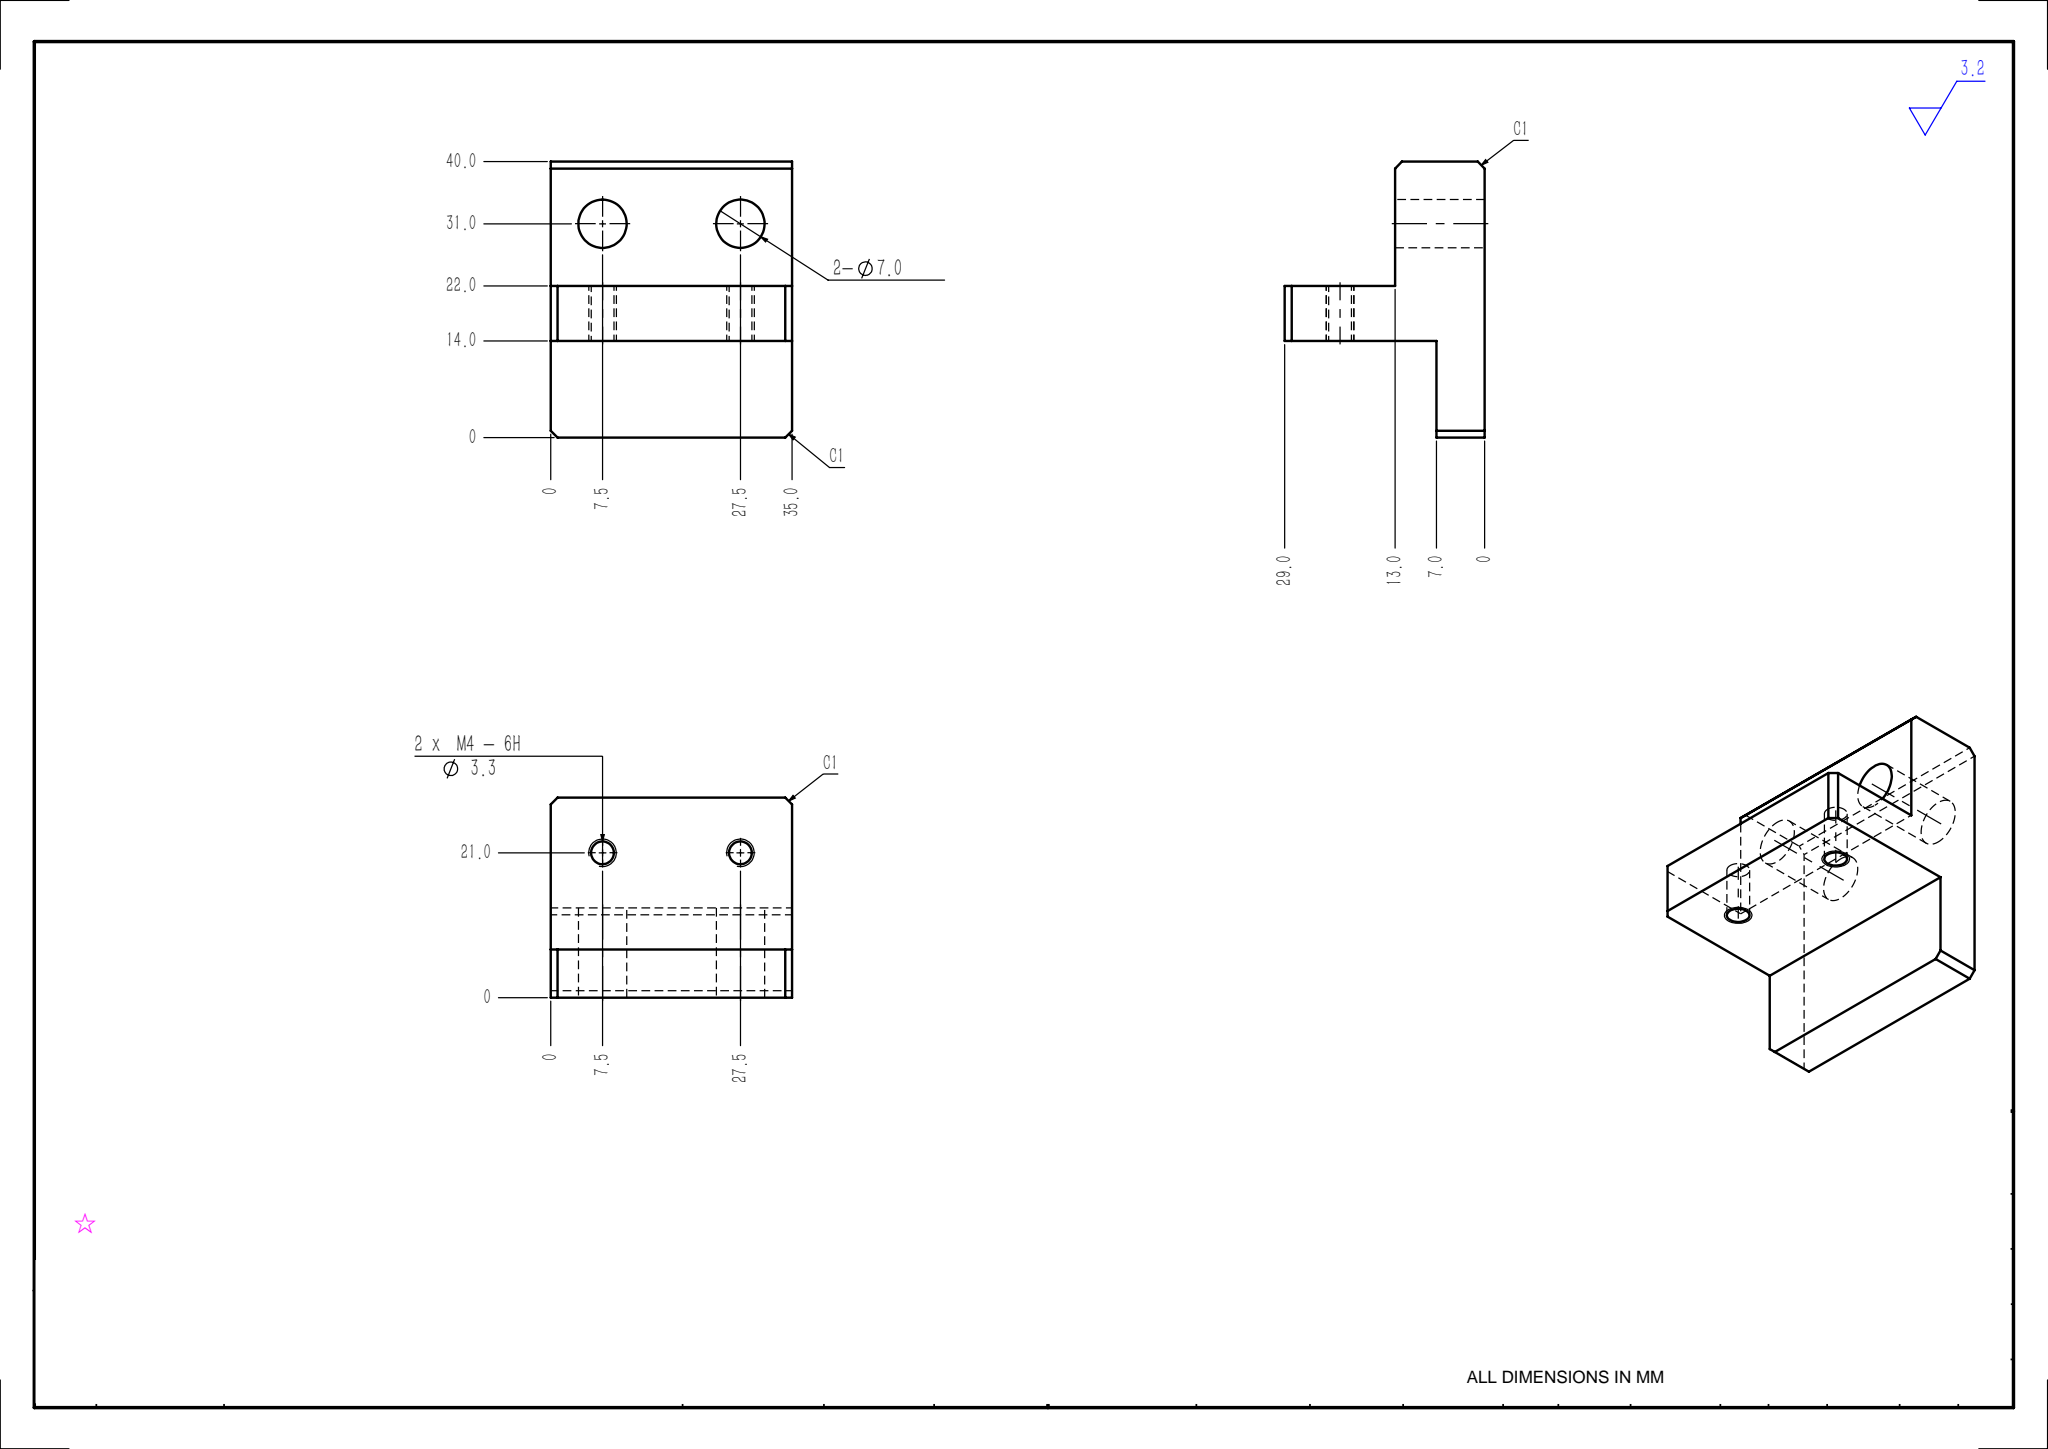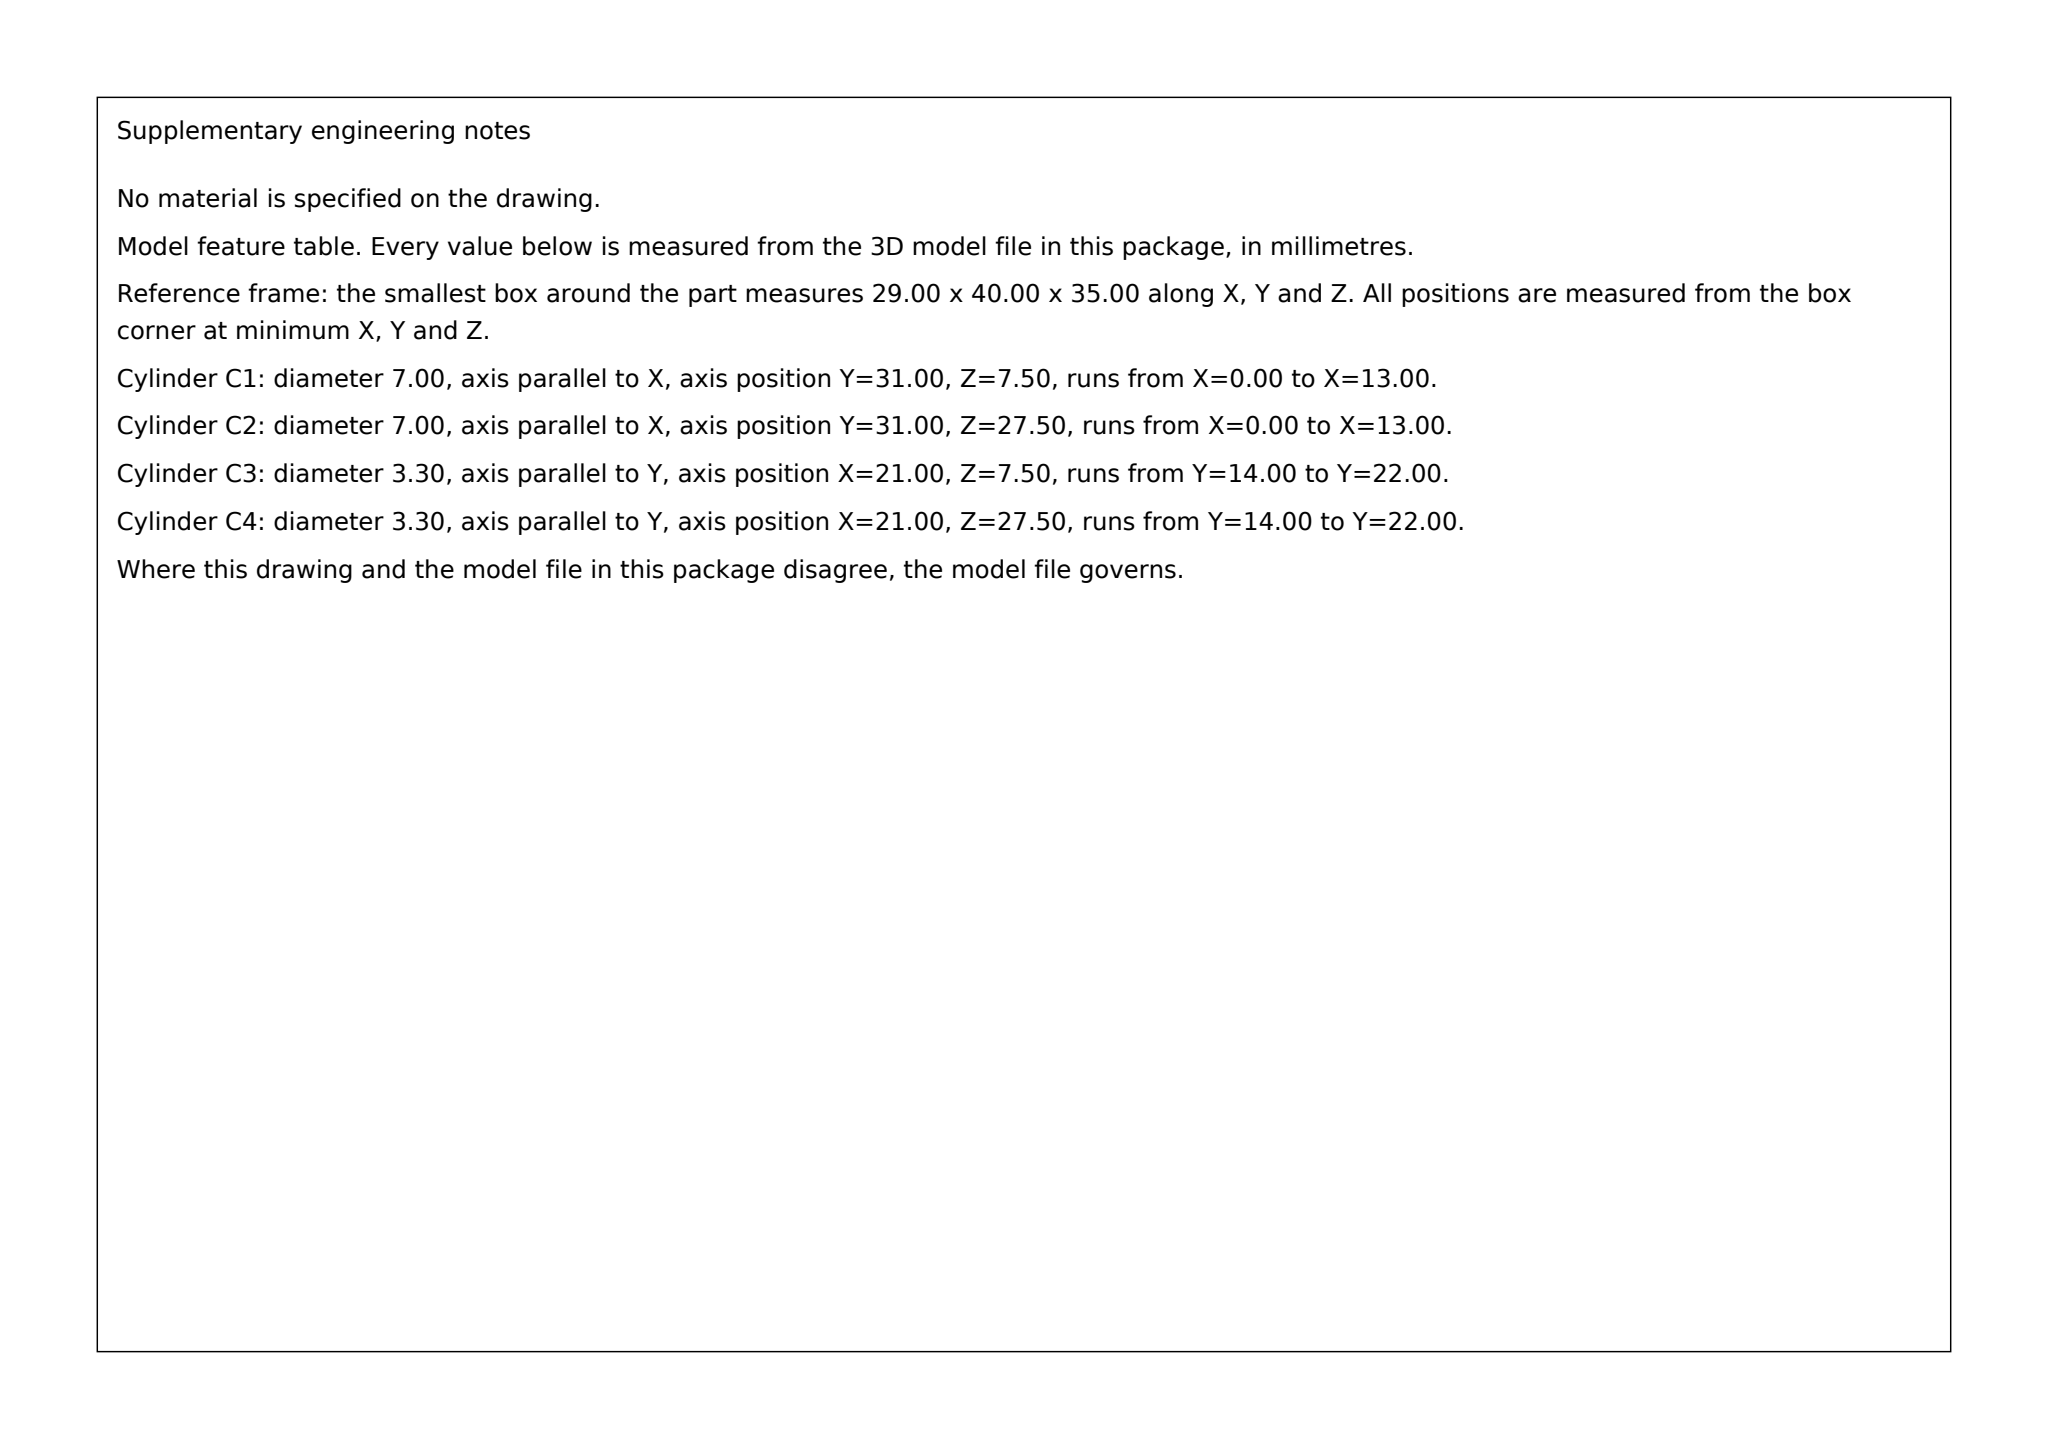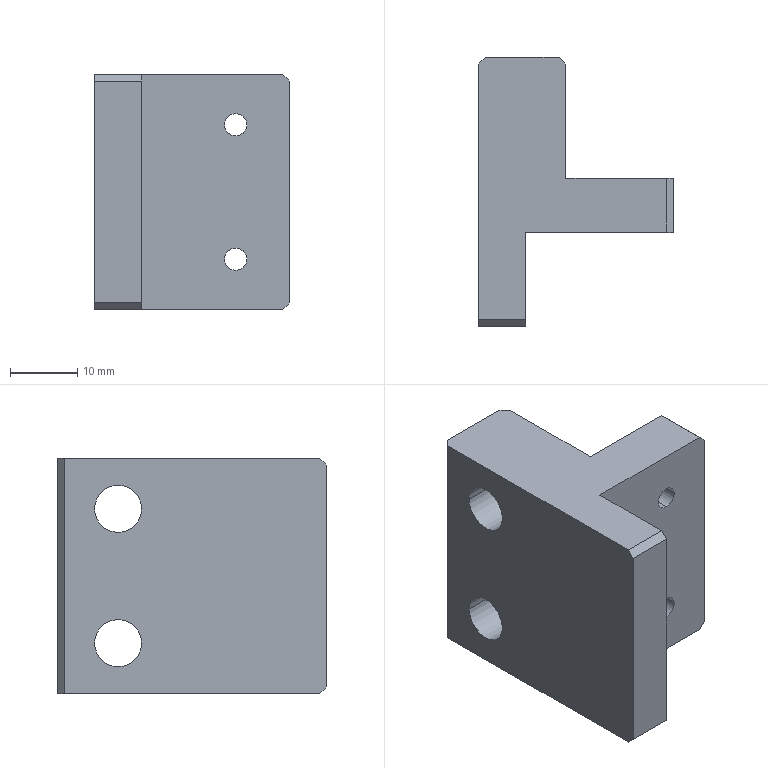Part | SolidWorks | mm | 1 solid | 24 faces | box 29 x 40 x 35 mm | volume 18553 mm3 | plane 16 | cylinder 8 | commonest cylinder face diameters 3.3 x4 7 x4
build123d program:
from build123d import *

# Parameters (mm, degrees)
SKETCH1_W           = 29
SKETCH1_H           = 40
BOSS_EXTRUDE1_DEPTH = 17.5
SKETCH2_W           = 22
SKETCH2_H           = 14
SKETCH2_W_2         = 16
SKETCH2_H_2         = 18
CUT_EXTRUDE1_DEPTH  = 43.84
SKETCH3_R           = 3.5
CUT_EXTRUDE2_DEPTH  = 32.02
M4_TAPPED_HOLE1_D   = 3.3
CHAMFER1_SIZE       = 1


with BuildPart() as part:
    # Sketch1 → Boss-Extrude1 (new, symmetric)
    with BuildSketch(Plane.XY):
        Rectangle(SKETCH1_W, SKETCH1_H)
    extrude(amount=BOSS_EXTRUDE1_DEPTH, both=True)

    # Sketch2 → Cut-Extrude1 (cut, through all)
    with BuildSketch(Plane.XY.offset(17.5)):
        with Locations((3.5, -13)):
            Rectangle(SKETCH2_W, SKETCH2_H)
        with Locations((6.5, 11)):
            Rectangle(SKETCH2_W_2, SKETCH2_H_2)
    extrude(amount=-CUT_EXTRUDE1_DEPTH, mode=Mode.SUBTRACT)

    # Sketch3 → Cut-Extrude2 (cut, through all)
    with BuildSketch(Plane(origin=(-1.5, 0, 0), x_dir=(0, 0, -1), z_dir=(1, 0, 0))):
        with Locations(Location((-10, 11, 0), (0, 0, 90))):
            Circle(SKETCH3_R)
        with Locations(Location((10, 11, 0), (0, 0, 270))):
            Circle(SKETCH3_R)
    extrude(amount=-CUT_EXTRUDE2_DEPTH, mode=Mode.SUBTRACT)

    # M4 Tapped Hole1 (through all)
    with Locations(Plane(origin=(0, -6, 0), x_dir=(-1, 0, 0), z_dir=(0, -1, 0))):
        with Locations((-6.5, 10), (-6.5, -10)):
            Hole(M4_TAPPED_HOLE1_D / 2)

    # Chamfer1
    chamfer1_edges = [part.edges().sort_by_distance(p)[0] for p in [
        (-11, -20, 17.5),
        (14.5, -2, -17.5),
        (14.5, -2, 17.5),
        (-1.5, 20, 0),
        (-11, -20, -17.5),
        (-14.5, 20, 0),
    ]]
    chamfer(chamfer1_edges, length=CHAMFER1_SIZE)


solid = part.part
STEP:
#1=CARTESIAN_POINT('',(6.5,2.,-8.35));
#2=VERTEX_POINT('',#1);
#3=CARTESIAN_POINT('',(6.5,2.,-11.65));
#4=VERTEX_POINT('',#3);
#5=CARTESIAN_POINT('',(6.5,2.,-10.));
#6=DIRECTION('',(0.,-1.,0.));
#7=DIRECTION('',(1.,0.,0.));
#8=AXIS2_PLACEMENT_3D('',#5,#6,#7);
#9=CIRCLE('',#8,1.65);
#10=EDGE_CURVE('',#2,#4,#9,.T.);
#11=ORIENTED_EDGE('',*,*,#10,.F.);
#12=CARTESIAN_POINT('',(6.5,-6.,-8.35));
#13=VERTEX_POINT('',#12);
#14=CARTESIAN_POINT('',(6.5,-6.,-8.35));
#15=DIRECTION('',(0.,-1.,0.));
#16=VECTOR('',#15,1000.);
#17=LINE('',#14,#16);
#18=EDGE_CURVE('',#2,#13,#17,.T.);
#19=ORIENTED_EDGE('',*,*,#18,.T.);
#20=CARTESIAN_POINT('',(6.5,-6.,-11.65));
#21=VERTEX_POINT('',#20);
#22=CARTESIAN_POINT('',(6.5,-6.,-10.));
#23=DIRECTION('',(0.,-1.,0.));
#24=DIRECTION('',(0.,0.,-1.));
#25=AXIS2_PLACEMENT_3D('',#22,#23,#24);
#26=CIRCLE('',#25,1.65);
#27=EDGE_CURVE('',#13,#21,#26,.T.);
#28=ORIENTED_EDGE('',*,*,#27,.T.);
#29=CARTESIAN_POINT('',(6.5,-6.,-11.65));
#30=DIRECTION('',(0.,-1.,0.));
#31=VECTOR('',#30,1000.);
#32=LINE('',#29,#31);
#33=EDGE_CURVE('',#4,#21,#32,.T.);
#34=ORIENTED_EDGE('',*,*,#33,.F.);
#35=EDGE_LOOP('',(#11,#19,#28,#34));
#36=FACE_OUTER_BOUND('',#35,.T.);
#37=CARTESIAN_POINT('',(6.5,-6.,-10.));
#38=DIRECTION('',(0.,-1.,0.));
#39=DIRECTION('',(0.,0.,-1.));
#40=AXIS2_PLACEMENT_3D('',#37,#38,#39);
#41=CYLINDRICAL_SURFACE('',#40,1.65);
#42=ADVANCED_FACE('',(#36),#41,.F.);
#43=CARTESIAN_POINT('',(6.5,2.,11.65));
#44=VERTEX_POINT('',#43);
#45=CARTESIAN_POINT('',(6.5,2.,8.35));
#46=VERTEX_POINT('',#45);
#47=CARTESIAN_POINT('',(6.5,2.,10.));
#48=DIRECTION('',(0.,-1.,0.));
#49=DIRECTION('',(1.,0.,0.));
#50=AXIS2_PLACEMENT_3D('',#47,#48,#49);
#51=CIRCLE('',#50,1.65);
#52=EDGE_CURVE('',#44,#46,#51,.T.);
#53=ORIENTED_EDGE('',*,*,#52,.F.);
#54=CARTESIAN_POINT('',(6.5,-6.,11.65));
#55=VERTEX_POINT('',#54);
#56=CARTESIAN_POINT('',(6.5,-6.,11.65));
#57=DIRECTION('',(0.,-1.,0.));
#58=VECTOR('',#57,1000.);
#59=LINE('',#56,#58);
#60=EDGE_CURVE('',#44,#55,#59,.T.);
#61=ORIENTED_EDGE('',*,*,#60,.T.);
#62=CARTESIAN_POINT('',(6.5,-6.,8.35));
#63=VERTEX_POINT('',#62);
#64=CARTESIAN_POINT('',(6.5,-6.,10.));
#65=DIRECTION('',(0.,-1.,0.));
#66=DIRECTION('',(0.,0.,-1.));
#67=AXIS2_PLACEMENT_3D('',#64,#65,#66);
#68=CIRCLE('',#67,1.65);
#69=EDGE_CURVE('',#55,#63,#68,.T.);
#70=ORIENTED_EDGE('',*,*,#69,.T.);
#71=CARTESIAN_POINT('',(6.5,-6.,8.35));
#72=DIRECTION('',(0.,-1.,0.));
#73=VECTOR('',#72,1000.);
#74=LINE('',#71,#73);
#75=EDGE_CURVE('',#46,#63,#74,.T.);
#76=ORIENTED_EDGE('',*,*,#75,.F.);
#77=EDGE_LOOP('',(#53,#61,#70,#76));
#78=FACE_OUTER_BOUND('',#77,.T.);
#79=CARTESIAN_POINT('',(6.5,-6.,10.));
#80=DIRECTION('',(0.,-1.,0.));
#81=DIRECTION('',(0.,0.,-1.));
#82=AXIS2_PLACEMENT_3D('',#79,#80,#81);
#83=CYLINDRICAL_SURFACE('',#82,1.65);
#84=ADVANCED_FACE('',(#78),#83,.F.);
#85=CARTESIAN_POINT('',(-14.5,7.5,10.));
#86=VERTEX_POINT('',#85);
#87=CARTESIAN_POINT('',(-14.5,14.5,10.));
#88=VERTEX_POINT('',#87);
#89=CARTESIAN_POINT('',(-14.5,11.,10.));
#90=DIRECTION('',(1.,0.,0.));
#91=DIRECTION('',(-0.,1.,0.));
#92=AXIS2_PLACEMENT_3D('',#89,#90,#91);
#93=CIRCLE('',#92,3.5);
#94=EDGE_CURVE('',#86,#88,#93,.T.);
#95=ORIENTED_EDGE('',*,*,#94,.F.);
#96=CARTESIAN_POINT('',(-1.5,7.5,10.));
#97=VERTEX_POINT('',#96);
#98=CARTESIAN_POINT('',(-14.5,7.5,10.));
#99=DIRECTION('',(1.,0.,0.));
#100=VECTOR('',#99,1000.);
#101=LINE('',#98,#100);
#102=EDGE_CURVE('',#86,#97,#101,.T.);
#103=ORIENTED_EDGE('',*,*,#102,.T.);
#104=CARTESIAN_POINT('',(-1.5,14.5,10.));
#105=VERTEX_POINT('',#104);
#106=CARTESIAN_POINT('',(-1.5,11.,10.));
#107=DIRECTION('',(1.,0.,0.));
#108=DIRECTION('',(-0.,1.,0.));
#109=AXIS2_PLACEMENT_3D('',#106,#107,#108);
#110=CIRCLE('',#109,3.5);
#111=EDGE_CURVE('',#97,#105,#110,.T.);
#112=ORIENTED_EDGE('',*,*,#111,.T.);
#113=CARTESIAN_POINT('',(-14.5,14.5,10.));
#114=DIRECTION('',(1.,0.,0.));
#115=VECTOR('',#114,1000.);
#116=LINE('',#113,#115);
#117=EDGE_CURVE('',#88,#105,#116,.T.);
#118=ORIENTED_EDGE('',*,*,#117,.F.);
#119=EDGE_LOOP('',(#95,#103,#112,#118));
#120=FACE_OUTER_BOUND('',#119,.T.);
#121=CARTESIAN_POINT('',(-14.5,11.,10.));
#122=DIRECTION('',(1.,0.,0.));
#123=DIRECTION('',(-0.,1.,0.));
#124=AXIS2_PLACEMENT_3D('',#121,#122,#123);
#125=CYLINDRICAL_SURFACE('',#124,3.5);
#126=ADVANCED_FACE('',(#120),#125,.F.);
#127=CARTESIAN_POINT('',(-14.5,7.5,-10.));
#128=VERTEX_POINT('',#127);
#129=CARTESIAN_POINT('',(-14.5,14.5,-10.));
#130=VERTEX_POINT('',#129);
#131=CARTESIAN_POINT('',(-14.5,11.,-10.));
#132=DIRECTION('',(1.,0.,0.));
#133=DIRECTION('',(0.,-1.,0.));
#134=AXIS2_PLACEMENT_3D('',#131,#132,#133);
#135=CIRCLE('',#134,3.5);
#136=EDGE_CURVE('',#128,#130,#135,.T.);
#137=ORIENTED_EDGE('',*,*,#136,.F.);
#138=CARTESIAN_POINT('',(-1.5,7.5,-10.));
#139=VERTEX_POINT('',#138);
#140=CARTESIAN_POINT('',(-14.5,7.5,-10.));
#141=DIRECTION('',(1.,0.,0.));
#142=VECTOR('',#141,1000.);
#143=LINE('',#140,#142);
#144=EDGE_CURVE('',#128,#139,#143,.T.);
#145=ORIENTED_EDGE('',*,*,#144,.T.);
#146=CARTESIAN_POINT('',(-1.5,14.5,-10.));
#147=VERTEX_POINT('',#146);
#148=CARTESIAN_POINT('',(-1.5,11.,-10.));
#149=DIRECTION('',(1.,0.,0.));
#150=DIRECTION('',(0.,-1.,0.));
#151=AXIS2_PLACEMENT_3D('',#148,#149,#150);
#152=CIRCLE('',#151,3.5);
#153=EDGE_CURVE('',#139,#147,#152,.T.);
#154=ORIENTED_EDGE('',*,*,#153,.T.);
#155=CARTESIAN_POINT('',(-14.5,14.5,-10.));
#156=DIRECTION('',(1.,0.,0.));
#157=VECTOR('',#156,1000.);
#158=LINE('',#155,#157);
#159=EDGE_CURVE('',#130,#147,#158,.T.);
#160=ORIENTED_EDGE('',*,*,#159,.F.);
#161=EDGE_LOOP('',(#137,#145,#154,#160));
#162=FACE_OUTER_BOUND('',#161,.T.);
#163=CARTESIAN_POINT('',(-14.5,11.,-10.));
#164=DIRECTION('',(1.,0.,0.));
#165=DIRECTION('',(-0.,1.,0.));
#166=AXIS2_PLACEMENT_3D('',#163,#164,#165);
#167=CYLINDRICAL_SURFACE('',#166,3.5);
#168=ADVANCED_FACE('',(#162),#167,.F.);
#169=CARTESIAN_POINT('',(14.5,-6.,-16.5));
#170=VERTEX_POINT('',#169);
#171=CARTESIAN_POINT('',(14.5,-6.,16.5));
#172=VERTEX_POINT('',#171);
#173=CARTESIAN_POINT('',(14.5,-6.,-17.5));
#174=DIRECTION('',(0.,0.,1.));
#175=VECTOR('',#174,1000.);
#176=LINE('',#173,#175);
#177=EDGE_CURVE('',#170,#172,#176,.T.);
#178=ORIENTED_EDGE('',*,*,#177,.F.);
#179=CARTESIAN_POINT('',(14.5,2.,-16.5));
#180=VERTEX_POINT('',#179);
#181=CARTESIAN_POINT('',(14.5,20.,-16.5));
#182=DIRECTION('',(-0.,1.,0.));
#183=VECTOR('',#182,1000.);
#184=LINE('',#181,#183);
#185=EDGE_CURVE('',#170,#180,#184,.T.);
#186=ORIENTED_EDGE('',*,*,#185,.T.);
#187=CARTESIAN_POINT('',(14.5,2.,16.5));
#188=VERTEX_POINT('',#187);
#189=CARTESIAN_POINT('',(14.5,2.,-17.5));
#190=DIRECTION('',(0.,0.,1.));
#191=VECTOR('',#190,1000.);
#192=LINE('',#189,#191);
#193=EDGE_CURVE('',#180,#188,#192,.T.);
#194=ORIENTED_EDGE('',*,*,#193,.T.);
#195=CARTESIAN_POINT('',(14.5,-6.,16.5));
#196=DIRECTION('',(0.,-1.,0.));
#197=VECTOR('',#196,1000.);
#198=LINE('',#195,#197);
#199=EDGE_CURVE('',#188,#172,#198,.T.);
#200=ORIENTED_EDGE('',*,*,#199,.T.);
#201=EDGE_LOOP('',(#178,#186,#194,#200));
#202=FACE_OUTER_BOUND('',#201,.T.);
#203=CARTESIAN_POINT('',(14.5,20.,17.5));
#204=DIRECTION('',(-1.,-0.,0.));
#205=DIRECTION('',(0.,-1.,0.));
#206=AXIS2_PLACEMENT_3D('',#203,#204,#205);
#207=PLANE('',#206);
#208=ADVANCED_FACE('',(#202),#207,.F.);
#209=CARTESIAN_POINT('',(-2.5,20.,17.5));
#210=VERTEX_POINT('',#209);
#211=CARTESIAN_POINT('',(-13.5,20.,17.5));
#212=VERTEX_POINT('',#211);
#213=CARTESIAN_POINT('',(-14.5,20.,17.5));
#214=DIRECTION('',(-1.,0.,0.));
#215=VECTOR('',#214,1000.);
#216=LINE('',#213,#215);
#217=EDGE_CURVE('',#210,#212,#216,.T.);
#218=ORIENTED_EDGE('',*,*,#217,.F.);
#219=CARTESIAN_POINT('',(-2.5,20.,-17.5));
#220=VERTEX_POINT('',#219);
#221=CARTESIAN_POINT('',(-2.5,20.,17.5));
#222=DIRECTION('',(0.,0.,-1.));
#223=VECTOR('',#222,1000.);
#224=LINE('',#221,#223);
#225=EDGE_CURVE('',#210,#220,#224,.T.);
#226=ORIENTED_EDGE('',*,*,#225,.T.);
#227=CARTESIAN_POINT('',(-13.5,20.,-17.5));
#228=VERTEX_POINT('',#227);
#229=CARTESIAN_POINT('',(-14.5,20.,-17.5));
#230=DIRECTION('',(-1.,0.,0.));
#231=VECTOR('',#230,1000.);
#232=LINE('',#229,#231);
#233=EDGE_CURVE('',#220,#228,#232,.T.);
#234=ORIENTED_EDGE('',*,*,#233,.T.);
#235=CARTESIAN_POINT('',(-13.5,20.,17.5));
#236=DIRECTION('',(0.,0.,1.));
#237=VECTOR('',#236,1000.);
#238=LINE('',#235,#237);
#239=EDGE_CURVE('',#228,#212,#238,.T.);
#240=ORIENTED_EDGE('',*,*,#239,.T.);
#241=EDGE_LOOP('',(#218,#226,#234,#240));
#242=FACE_OUTER_BOUND('',#241,.T.);
#243=CARTESIAN_POINT('',(-14.5,20.,17.5));
#244=DIRECTION('',(0.,-1.,0.));
#245=DIRECTION('',(0.,0.,-1.));
#246=AXIS2_PLACEMENT_3D('',#243,#244,#245);
#247=PLANE('',#246);
#248=ADVANCED_FACE('',(#242),#247,.F.);
#249=CARTESIAN_POINT('',(-14.5,11.,10.));
#250=DIRECTION('',(1.,0.,0.));
#251=DIRECTION('',(-0.,1.,0.));
#252=AXIS2_PLACEMENT_3D('',#249,#250,#251);
#253=CIRCLE('',#252,3.5);
#254=EDGE_CURVE('',#88,#86,#253,.T.);
#255=ORIENTED_EDGE('',*,*,#254,.T.);
#256=ORIENTED_EDGE('',*,*,#94,.T.);
#257=EDGE_LOOP('',(#255,#256));
#258=FACE_BOUND('',#257,.T.);
#259=CARTESIAN_POINT('',(-14.5,11.,-10.));
#260=DIRECTION('',(1.,0.,0.));
#261=DIRECTION('',(0.,-1.,0.));
#262=AXIS2_PLACEMENT_3D('',#259,#260,#261);
#263=CIRCLE('',#262,3.5);
#264=EDGE_CURVE('',#130,#128,#263,.T.);
#265=ORIENTED_EDGE('',*,*,#264,.T.);
#266=ORIENTED_EDGE('',*,*,#136,.T.);
#267=EDGE_LOOP('',(#265,#266));
#268=FACE_BOUND('',#267,.T.);
#269=CARTESIAN_POINT('',(-14.5,19.,-17.5));
#270=VERTEX_POINT('',#269);
#271=CARTESIAN_POINT('',(-14.5,-19.,-17.5));
#272=VERTEX_POINT('',#271);
#273=CARTESIAN_POINT('',(-14.5,20.,-17.5));
#274=DIRECTION('',(0.,-1.,0.));
#275=VECTOR('',#274,1000.);
#276=LINE('',#273,#275);
#277=EDGE_CURVE('',#270,#272,#276,.T.);
#278=ORIENTED_EDGE('',*,*,#277,.T.);
#279=CARTESIAN_POINT('',(-14.5,-20.,-16.5));
#280=VERTEX_POINT('',#279);
#281=CARTESIAN_POINT('',(-14.5,-20.,-16.5));
#282=DIRECTION('',(0.,-0.7071,0.7071));
#283=VECTOR('',#282,1000.);
#284=LINE('',#281,#283);
#285=EDGE_CURVE('',#272,#280,#284,.T.);
#286=ORIENTED_EDGE('',*,*,#285,.T.);
#287=CARTESIAN_POINT('',(-14.5,-20.,16.5));
#288=VERTEX_POINT('',#287);
#289=CARTESIAN_POINT('',(-14.5,-20.,17.5));
#290=DIRECTION('',(0.,0.,-1.));
#291=VECTOR('',#290,1000.);
#292=LINE('',#289,#291);
#293=EDGE_CURVE('',#288,#280,#292,.T.);
#294=ORIENTED_EDGE('',*,*,#293,.F.);
#295=CARTESIAN_POINT('',(-14.5,-19.,17.5));
#296=VERTEX_POINT('',#295);
#297=CARTESIAN_POINT('',(-14.5,-19.,17.5));
#298=DIRECTION('',(-0.,0.7071,0.7071));
#299=VECTOR('',#298,1000.);
#300=LINE('',#297,#299);
#301=EDGE_CURVE('',#288,#296,#300,.T.);
#302=ORIENTED_EDGE('',*,*,#301,.T.);
#303=CARTESIAN_POINT('',(-14.5,19.,17.5));
#304=VERTEX_POINT('',#303);
#305=CARTESIAN_POINT('',(-14.5,20.,17.5));
#306=DIRECTION('',(0.,-1.,0.));
#307=VECTOR('',#306,1000.);
#308=LINE('',#305,#307);
#309=EDGE_CURVE('',#304,#296,#308,.T.);
#310=ORIENTED_EDGE('',*,*,#309,.F.);
#311=CARTESIAN_POINT('',(-14.5,19.,17.5));
#312=DIRECTION('',(0.,0.,-1.));
#313=VECTOR('',#312,1000.);
#314=LINE('',#311,#313);
#315=EDGE_CURVE('',#304,#270,#314,.T.);
#316=ORIENTED_EDGE('',*,*,#315,.T.);
#317=EDGE_LOOP('',(#278,#286,#294,#302,#310,#316));
#318=FACE_OUTER_BOUND('',#317,.T.);
#319=CARTESIAN_POINT('',(-14.5,20.,17.5));
#320=DIRECTION('',(1.,0.,0.));
#321=DIRECTION('',(-0.,1.,0.));
#322=AXIS2_PLACEMENT_3D('',#319,#320,#321);
#323=PLANE('',#322);
#324=ADVANCED_FACE('',(#258,#268,#318),#323,.F.);
#325=ORIENTED_EDGE('',*,*,#293,.T.);
#326=CARTESIAN_POINT('',(-7.5,-20.,-16.5));
#327=VERTEX_POINT('',#326);
#328=CARTESIAN_POINT('',(-14.5,-20.,-16.5));
#329=DIRECTION('',(1.,0.,0.));
#330=VECTOR('',#329,1000.);
#331=LINE('',#328,#330);
#332=EDGE_CURVE('',#280,#327,#331,.T.);
#333=ORIENTED_EDGE('',*,*,#332,.T.);
#334=CARTESIAN_POINT('',(-7.5,-20.,16.5));
#335=VERTEX_POINT('',#334);
#336=CARTESIAN_POINT('',(-7.5,-20.,-17.5));
#337=DIRECTION('',(0.,0.,1.));
#338=VECTOR('',#337,1000.);
#339=LINE('',#336,#338);
#340=EDGE_CURVE('',#327,#335,#339,.T.);
#341=ORIENTED_EDGE('',*,*,#340,.T.);
#342=CARTESIAN_POINT('',(-14.5,-20.,16.5));
#343=DIRECTION('',(-1.,0.,0.));
#344=VECTOR('',#343,1000.);
#345=LINE('',#342,#344);
#346=EDGE_CURVE('',#335,#288,#345,.T.);
#347=ORIENTED_EDGE('',*,*,#346,.T.);
#348=EDGE_LOOP('',(#325,#333,#341,#347));
#349=FACE_OUTER_BOUND('',#348,.T.);
#350=CARTESIAN_POINT('',(-14.5,-20.,17.5));
#351=DIRECTION('',(0.,1.,0.));
#352=DIRECTION('',(0.,0.,1.));
#353=AXIS2_PLACEMENT_3D('',#350,#351,#352);
#354=PLANE('',#353);
#355=ADVANCED_FACE('',(#349),#354,.F.);
#356=ORIENTED_EDGE('',*,*,#309,.T.);
#357=CARTESIAN_POINT('',(-7.5,-19.,17.5));
#358=VERTEX_POINT('',#357);
#359=CARTESIAN_POINT('',(-7.5,-19.,17.5));
#360=DIRECTION('',(1.,0.,0.));
#361=VECTOR('',#360,1000.);
#362=LINE('',#359,#361);
#363=EDGE_CURVE('',#296,#358,#362,.T.);
#364=ORIENTED_EDGE('',*,*,#363,.T.);
#365=CARTESIAN_POINT('',(-7.5,-6.,17.5));
#366=VERTEX_POINT('',#365);
#367=CARTESIAN_POINT('',(-7.5,-20.,17.5));
#368=DIRECTION('',(0.,-1.,0.));
#369=VECTOR('',#368,1000.);
#370=LINE('',#367,#369);
#371=EDGE_CURVE('',#366,#358,#370,.T.);
#372=ORIENTED_EDGE('',*,*,#371,.F.);
#373=CARTESIAN_POINT('',(13.5,-6.,17.5));
#374=VERTEX_POINT('',#373);
#375=CARTESIAN_POINT('',(14.5,-6.,17.5));
#376=DIRECTION('',(-1.,-0.,0.));
#377=VECTOR('',#376,1000.);
#378=LINE('',#375,#377);
#379=EDGE_CURVE('',#374,#366,#378,.T.);
#380=ORIENTED_EDGE('',*,*,#379,.F.);
#381=CARTESIAN_POINT('',(13.5,2.,17.5));
#382=VERTEX_POINT('',#381);
#383=CARTESIAN_POINT('',(13.5,2.,17.5));
#384=DIRECTION('',(-0.,1.,0.));
#385=VECTOR('',#384,1000.);
#386=LINE('',#383,#385);
#387=EDGE_CURVE('',#374,#382,#386,.T.);
#388=ORIENTED_EDGE('',*,*,#387,.T.);
#389=CARTESIAN_POINT('',(-1.5,2.,17.5));
#390=VERTEX_POINT('',#389);
#391=CARTESIAN_POINT('',(14.5,2.,17.5));
#392=DIRECTION('',(1.,0.,0.));
#393=VECTOR('',#392,1000.);
#394=LINE('',#391,#393);
#395=EDGE_CURVE('',#390,#382,#394,.T.);
#396=ORIENTED_EDGE('',*,*,#395,.F.);
#397=CARTESIAN_POINT('',(-1.5,19.,17.5));
#398=VERTEX_POINT('',#397);
#399=CARTESIAN_POINT('',(-1.5,20.,17.5));
#400=DIRECTION('',(0.,-1.,0.));
#401=VECTOR('',#400,1000.);
#402=LINE('',#399,#401);
#403=EDGE_CURVE('',#398,#390,#402,.T.);
#404=ORIENTED_EDGE('',*,*,#403,.F.);
#405=CARTESIAN_POINT('',(8.75,8.75,17.5));
#406=DIRECTION('',(-0.7071,0.7071,0.));
#407=VECTOR('',#406,1000.);
#408=LINE('',#405,#407);
#409=EDGE_CURVE('',#398,#210,#408,.T.);
#410=ORIENTED_EDGE('',*,*,#409,.T.);
#411=ORIENTED_EDGE('',*,*,#217,.T.);
#412=CARTESIAN_POINT('',(-16.75,16.75,17.5));
#413=DIRECTION('',(-0.7071,-0.7071,0.));
#414=VECTOR('',#413,1000.);
#415=LINE('',#412,#414);
#416=EDGE_CURVE('',#212,#304,#415,.T.);
#417=ORIENTED_EDGE('',*,*,#416,.T.);
#418=EDGE_LOOP('',(#356,#364,#372,#380,#388,#396,#404,#410,#411,#417));
#419=FACE_OUTER_BOUND('',#418,.T.);
#420=CARTESIAN_POINT('',(0.,0.,17.5));
#421=DIRECTION('',(0.,0.,1.));
#422=DIRECTION('',(1.,0.,0.));
#423=AXIS2_PLACEMENT_3D('',#420,#421,#422);
#424=PLANE('',#423);
#425=ADVANCED_FACE('',(#419),#424,.T.);
#426=CARTESIAN_POINT('',(-7.5,-6.,-17.5));
#427=VERTEX_POINT('',#426);
#428=CARTESIAN_POINT('',(-7.5,-19.,-17.5));
#429=VERTEX_POINT('',#428);
#430=CARTESIAN_POINT('',(-7.5,-20.,-17.5));
#431=DIRECTION('',(0.,-1.,0.));
#432=VECTOR('',#431,1000.);
#433=LINE('',#430,#432);
#434=EDGE_CURVE('',#427,#429,#433,.T.);
#435=ORIENTED_EDGE('',*,*,#434,.T.);
#436=CARTESIAN_POINT('',(0.,-19.,-17.5));
#437=DIRECTION('',(-1.,0.,0.));
#438=VECTOR('',#437,1000.);
#439=LINE('',#436,#438);
#440=EDGE_CURVE('',#429,#272,#439,.T.);
#441=ORIENTED_EDGE('',*,*,#440,.T.);
#442=ORIENTED_EDGE('',*,*,#277,.F.);
#443=CARTESIAN_POINT('',(-14.5,19.,-17.5));
#444=DIRECTION('',(0.7071,0.7071,0.));
#445=VECTOR('',#444,1000.);
#446=LINE('',#443,#445);
#447=EDGE_CURVE('',#270,#228,#446,.T.);
#448=ORIENTED_EDGE('',*,*,#447,.T.);
#449=ORIENTED_EDGE('',*,*,#233,.F.);
#450=CARTESIAN_POINT('',(-1.5,19.,-17.5));
#451=VERTEX_POINT('',#450);
#452=CARTESIAN_POINT('',(-1.5,19.,-17.5));
#453=DIRECTION('',(0.7071,-0.7071,0.));
#454=VECTOR('',#453,1000.);
#455=LINE('',#452,#454);
#456=EDGE_CURVE('',#220,#451,#455,.T.);
#457=ORIENTED_EDGE('',*,*,#456,.T.);
#458=CARTESIAN_POINT('',(-1.5,2.,-17.5));
#459=VERTEX_POINT('',#458);
#460=CARTESIAN_POINT('',(-1.5,20.,-17.5));
#461=DIRECTION('',(0.,-1.,0.));
#462=VECTOR('',#461,1000.);
#463=LINE('',#460,#462);
#464=EDGE_CURVE('',#451,#459,#463,.T.);
#465=ORIENTED_EDGE('',*,*,#464,.T.);
#466=CARTESIAN_POINT('',(13.5,2.,-17.5));
#467=VERTEX_POINT('',#466);
#468=CARTESIAN_POINT('',(14.5,2.,-17.5));
#469=DIRECTION('',(1.,0.,0.));
#470=VECTOR('',#469,1000.);
#471=LINE('',#468,#470);
#472=EDGE_CURVE('',#459,#467,#471,.T.);
#473=ORIENTED_EDGE('',*,*,#472,.T.);
#474=CARTESIAN_POINT('',(13.5,-6.,-17.5));
#475=VERTEX_POINT('',#474);
#476=CARTESIAN_POINT('',(13.5,0.,-17.5));
#477=DIRECTION('',(0.,-1.,0.));
#478=VECTOR('',#477,1000.);
#479=LINE('',#476,#478);
#480=EDGE_CURVE('',#467,#475,#479,.T.);
#481=ORIENTED_EDGE('',*,*,#480,.T.);
#482=CARTESIAN_POINT('',(14.5,-6.,-17.5));
#483=DIRECTION('',(-1.,-0.,0.));
#484=VECTOR('',#483,1000.);
#485=LINE('',#482,#484);
#486=EDGE_CURVE('',#475,#427,#485,.T.);
#487=ORIENTED_EDGE('',*,*,#486,.T.);
#488=EDGE_LOOP('',(#435,#441,#442,#448,#449,#457,#465,#473,#481,#487));
#489=FACE_OUTER_BOUND('',#488,.T.);
#490=CARTESIAN_POINT('',(0.,0.,-17.5));
#491=DIRECTION('',(0.,0.,1.));
#492=DIRECTION('',(1.,0.,0.));
#493=AXIS2_PLACEMENT_3D('',#490,#491,#492);
#494=PLANE('',#493);
#495=ADVANCED_FACE('',(#489),#494,.F.);
#496=CARTESIAN_POINT('',(6.5,2.,-10.));
#497=DIRECTION('',(0.,-1.,0.));
#498=DIRECTION('',(1.,0.,0.));
#499=AXIS2_PLACEMENT_3D('',#496,#497,#498);
#500=CIRCLE('',#499,1.65);
#501=EDGE_CURVE('',#4,#2,#500,.T.);
#502=ORIENTED_EDGE('',*,*,#501,.T.);
#503=ORIENTED_EDGE('',*,*,#10,.T.);
#504=EDGE_LOOP('',(#502,#503));
#505=FACE_BOUND('',#504,.T.);
#506=CARTESIAN_POINT('',(6.5,2.,10.));
#507=DIRECTION('',(0.,-1.,0.));
#508=DIRECTION('',(1.,0.,0.));
#509=AXIS2_PLACEMENT_3D('',#506,#507,#508);
#510=CIRCLE('',#509,1.65);
#511=EDGE_CURVE('',#46,#44,#510,.T.);
#512=ORIENTED_EDGE('',*,*,#511,.T.);
#513=ORIENTED_EDGE('',*,*,#52,.T.);
#514=EDGE_LOOP('',(#512,#513));
#515=FACE_BOUND('',#514,.T.);
#516=ORIENTED_EDGE('',*,*,#193,.F.);
#517=CARTESIAN_POINT('',(14.5,2.,-16.5));
#518=DIRECTION('',(-0.7071,-0.,-0.7071));
#519=VECTOR('',#518,1000.);
#520=LINE('',#517,#519);
#521=EDGE_CURVE('',#180,#467,#520,.T.);
#522=ORIENTED_EDGE('',*,*,#521,.T.);
#523=ORIENTED_EDGE('',*,*,#472,.F.);
#524=CARTESIAN_POINT('',(-1.5,2.,-17.5));
#525=DIRECTION('',(0.,0.,1.));
#526=VECTOR('',#525,1000.);
#527=LINE('',#524,#526);
#528=EDGE_CURVE('',#459,#390,#527,.T.);
#529=ORIENTED_EDGE('',*,*,#528,.T.);
#530=ORIENTED_EDGE('',*,*,#395,.T.);
#531=CARTESIAN_POINT('',(13.5,2.,17.5));
#532=DIRECTION('',(0.7071,0.,-0.7071));
#533=VECTOR('',#532,1000.);
#534=LINE('',#531,#533);
#535=EDGE_CURVE('',#382,#188,#534,.T.);
#536=ORIENTED_EDGE('',*,*,#535,.T.);
#537=EDGE_LOOP('',(#516,#522,#523,#529,#530,#536));
#538=FACE_OUTER_BOUND('',#537,.T.);
#539=CARTESIAN_POINT('',(14.5,2.,-17.5));
#540=DIRECTION('',(0.,-1.,0.));
#541=DIRECTION('',(1.,0.,0.));
#542=AXIS2_PLACEMENT_3D('',#539,#540,#541);
#543=PLANE('',#542);
#544=ADVANCED_FACE('',(#505,#515,#538),#543,.F.);
#545=CARTESIAN_POINT('',(-1.5,11.,10.));
#546=DIRECTION('',(1.,0.,0.));
#547=DIRECTION('',(-0.,1.,0.));
#548=AXIS2_PLACEMENT_3D('',#545,#546,#547);
#549=CIRCLE('',#548,3.5);
#550=EDGE_CURVE('',#105,#97,#549,.T.);
#551=ORIENTED_EDGE('',*,*,#550,.F.);
#552=ORIENTED_EDGE('',*,*,#111,.F.);
#553=EDGE_LOOP('',(#551,#552));
#554=FACE_BOUND('',#553,.T.);
#555=CARTESIAN_POINT('',(-1.5,11.,-10.));
#556=DIRECTION('',(1.,0.,0.));
#557=DIRECTION('',(0.,-1.,0.));
#558=AXIS2_PLACEMENT_3D('',#555,#556,#557);
#559=CIRCLE('',#558,3.5);
#560=EDGE_CURVE('',#147,#139,#559,.T.);
#561=ORIENTED_EDGE('',*,*,#560,.F.);
#562=ORIENTED_EDGE('',*,*,#153,.F.);
#563=EDGE_LOOP('',(#561,#562));
#564=FACE_BOUND('',#563,.T.);
#565=ORIENTED_EDGE('',*,*,#464,.F.);
#566=CARTESIAN_POINT('',(-1.5,19.,-17.5));
#567=DIRECTION('',(0.,0.,1.));
#568=VECTOR('',#567,1000.);
#569=LINE('',#566,#568);
#570=EDGE_CURVE('',#451,#398,#569,.T.);
#571=ORIENTED_EDGE('',*,*,#570,.T.);
#572=ORIENTED_EDGE('',*,*,#403,.T.);
#573=ORIENTED_EDGE('',*,*,#528,.F.);
#574=EDGE_LOOP('',(#565,#571,#572,#573));
#575=FACE_OUTER_BOUND('',#574,.T.);
#576=CARTESIAN_POINT('',(-1.5,20.,-17.5));
#577=DIRECTION('',(-1.,-0.,0.));
#578=DIRECTION('',(0.,-1.,0.));
#579=AXIS2_PLACEMENT_3D('',#576,#577,#578);
#580=PLANE('',#579);
#581=ADVANCED_FACE('',(#554,#564,#575),#580,.F.);
#582=ORIENTED_EDGE('',*,*,#340,.F.);
#583=CARTESIAN_POINT('',(-7.5,-20.,-16.5));
#584=DIRECTION('',(0.,0.7071,-0.7071));
#585=VECTOR('',#584,1000.);
#586=LINE('',#583,#585);
#587=EDGE_CURVE('',#327,#429,#586,.T.);
#588=ORIENTED_EDGE('',*,*,#587,.T.);
#589=ORIENTED_EDGE('',*,*,#434,.F.);
#590=CARTESIAN_POINT('',(-7.5,-6.,-17.5));
#591=DIRECTION('',(0.,0.,1.));
#592=VECTOR('',#591,1000.);
#593=LINE('',#590,#592);
#594=EDGE_CURVE('',#427,#366,#593,.T.);
#595=ORIENTED_EDGE('',*,*,#594,.T.);
#596=ORIENTED_EDGE('',*,*,#371,.T.);
#597=CARTESIAN_POINT('',(-7.5,-19.,17.5));
#598=DIRECTION('',(0.,-0.7071,-0.7071));
#599=VECTOR('',#598,1000.);
#600=LINE('',#597,#599);
#601=EDGE_CURVE('',#358,#335,#600,.T.);
#602=ORIENTED_EDGE('',*,*,#601,.T.);
#603=EDGE_LOOP('',(#582,#588,#589,#595,#596,#602));
#604=FACE_OUTER_BOUND('',#603,.T.);
#605=CARTESIAN_POINT('',(-7.5,-20.,-17.5));
#606=DIRECTION('',(-1.,0.,0.));
#607=DIRECTION('',(0.,0.,1.));
#608=AXIS2_PLACEMENT_3D('',#605,#606,#607);
#609=PLANE('',#608);
#610=ADVANCED_FACE('',(#604),#609,.F.);
#611=CARTESIAN_POINT('',(6.5,-6.,-10.));
#612=DIRECTION('',(0.,-1.,0.));
#613=DIRECTION('',(0.,0.,-1.));
#614=AXIS2_PLACEMENT_3D('',#611,#612,#613);
#615=CIRCLE('',#614,1.65);
#616=EDGE_CURVE('',#21,#13,#615,.T.);
#617=ORIENTED_EDGE('',*,*,#616,.F.);
#618=ORIENTED_EDGE('',*,*,#27,.F.);
#619=EDGE_LOOP('',(#617,#618));
#620=FACE_BOUND('',#619,.T.);
#621=CARTESIAN_POINT('',(6.5,-6.,10.));
#622=DIRECTION('',(0.,-1.,0.));
#623=DIRECTION('',(0.,0.,-1.));
#624=AXIS2_PLACEMENT_3D('',#621,#622,#623);
#625=CIRCLE('',#624,1.65);
#626=EDGE_CURVE('',#63,#55,#625,.T.);
#627=ORIENTED_EDGE('',*,*,#626,.F.);
#628=ORIENTED_EDGE('',*,*,#69,.F.);
#629=EDGE_LOOP('',(#627,#628));
#630=FACE_BOUND('',#629,.T.);
#631=ORIENTED_EDGE('',*,*,#486,.F.);
#632=CARTESIAN_POINT('',(14.5,-6.,-16.5));
#633=DIRECTION('',(0.7071,0.,0.7071));
#634=VECTOR('',#633,1000.);
#635=LINE('',#632,#634);
#636=EDGE_CURVE('',#475,#170,#635,.T.);
#637=ORIENTED_EDGE('',*,*,#636,.T.);
#638=ORIENTED_EDGE('',*,*,#177,.T.);
#639=CARTESIAN_POINT('',(13.5,-6.,17.5));
#640=DIRECTION('',(-0.7071,-0.,0.7071));
#641=VECTOR('',#640,1000.);
#642=LINE('',#639,#641);
#643=EDGE_CURVE('',#172,#374,#642,.T.);
#644=ORIENTED_EDGE('',*,*,#643,.T.);
#645=ORIENTED_EDGE('',*,*,#379,.T.);
#646=ORIENTED_EDGE('',*,*,#594,.F.);
#647=EDGE_LOOP('',(#631,#637,#638,#644,#645,#646));
#648=FACE_OUTER_BOUND('',#647,.T.);
#649=CARTESIAN_POINT('',(14.5,-6.,-17.5));
#650=DIRECTION('',(-0.,1.,0.));
#651=DIRECTION('',(-1.,-0.,0.));
#652=AXIS2_PLACEMENT_3D('',#649,#650,#651);
#653=PLANE('',#652);
#654=ADVANCED_FACE('',(#620,#630,#648),#653,.F.);
#655=ORIENTED_EDGE('',*,*,#144,.F.);
#656=ORIENTED_EDGE('',*,*,#264,.F.);
#657=ORIENTED_EDGE('',*,*,#159,.T.);
#658=ORIENTED_EDGE('',*,*,#560,.T.);
#659=EDGE_LOOP('',(#655,#656,#657,#658));
#660=FACE_OUTER_BOUND('',#659,.T.);
#661=CARTESIAN_POINT('',(-14.5,11.,-10.));
#662=DIRECTION('',(1.,0.,0.));
#663=DIRECTION('',(-0.,1.,0.));
#664=AXIS2_PLACEMENT_3D('',#661,#662,#663);
#665=CYLINDRICAL_SURFACE('',#664,3.5);
#666=ADVANCED_FACE('',(#660),#665,.F.);
#667=ORIENTED_EDGE('',*,*,#102,.F.);
#668=ORIENTED_EDGE('',*,*,#254,.F.);
#669=ORIENTED_EDGE('',*,*,#117,.T.);
#670=ORIENTED_EDGE('',*,*,#550,.T.);
#671=EDGE_LOOP('',(#667,#668,#669,#670));
#672=FACE_OUTER_BOUND('',#671,.T.);
#673=CARTESIAN_POINT('',(-14.5,11.,10.));
#674=DIRECTION('',(1.,0.,0.));
#675=DIRECTION('',(-0.,1.,0.));
#676=AXIS2_PLACEMENT_3D('',#673,#674,#675);
#677=CYLINDRICAL_SURFACE('',#676,3.5);
#678=ADVANCED_FACE('',(#672),#677,.F.);
#679=ORIENTED_EDGE('',*,*,#60,.F.);
#680=ORIENTED_EDGE('',*,*,#511,.F.);
#681=ORIENTED_EDGE('',*,*,#75,.T.);
#682=ORIENTED_EDGE('',*,*,#626,.T.);
#683=EDGE_LOOP('',(#679,#680,#681,#682));
#684=FACE_OUTER_BOUND('',#683,.T.);
#685=CARTESIAN_POINT('',(6.5,-6.,10.));
#686=DIRECTION('',(0.,-1.,0.));
#687=DIRECTION('',(0.,0.,-1.));
#688=AXIS2_PLACEMENT_3D('',#685,#686,#687);
#689=CYLINDRICAL_SURFACE('',#688,1.65);
#690=ADVANCED_FACE('',(#684),#689,.F.);
#691=ORIENTED_EDGE('',*,*,#18,.F.);
#692=ORIENTED_EDGE('',*,*,#501,.F.);
#693=ORIENTED_EDGE('',*,*,#33,.T.);
#694=ORIENTED_EDGE('',*,*,#616,.T.);
#695=EDGE_LOOP('',(#691,#692,#693,#694));
#696=FACE_OUTER_BOUND('',#695,.T.);
#697=CARTESIAN_POINT('',(6.5,-6.,-10.));
#698=DIRECTION('',(0.,-1.,0.));
#699=DIRECTION('',(0.,0.,-1.));
#700=AXIS2_PLACEMENT_3D('',#697,#698,#699);
#701=CYLINDRICAL_SURFACE('',#700,1.65);
#702=ADVANCED_FACE('',(#696),#701,.F.);
#703=ORIENTED_EDGE('',*,*,#285,.F.);
#704=ORIENTED_EDGE('',*,*,#440,.F.);
#705=ORIENTED_EDGE('',*,*,#587,.F.);
#706=ORIENTED_EDGE('',*,*,#332,.F.);
#707=EDGE_LOOP('',(#703,#704,#705,#706));
#708=FACE_OUTER_BOUND('',#707,.T.);
#709=CARTESIAN_POINT('',(-14.5,-20.,-16.5));
#710=DIRECTION('',(0.,0.7071,0.7071));
#711=DIRECTION('',(1.,0.,0.));
#712=AXIS2_PLACEMENT_3D('',#709,#710,#711);
#713=PLANE('',#712);
#714=ADVANCED_FACE('',(#708),#713,.F.);
#715=ORIENTED_EDGE('',*,*,#301,.F.);
#716=ORIENTED_EDGE('',*,*,#346,.F.);
#717=ORIENTED_EDGE('',*,*,#601,.F.);
#718=ORIENTED_EDGE('',*,*,#363,.F.);
#719=EDGE_LOOP('',(#715,#716,#717,#718));
#720=FACE_OUTER_BOUND('',#719,.T.);
#721=CARTESIAN_POINT('',(0.,-19.,17.5));
#722=DIRECTION('',(0.,-0.7071,0.7071));
#723=DIRECTION('',(-1.,0.,0.));
#724=AXIS2_PLACEMENT_3D('',#721,#722,#723);
#725=PLANE('',#724);
#726=ADVANCED_FACE('',(#720),#725,.T.);
#727=ORIENTED_EDGE('',*,*,#636,.F.);
#728=ORIENTED_EDGE('',*,*,#480,.F.);
#729=ORIENTED_EDGE('',*,*,#521,.F.);
#730=ORIENTED_EDGE('',*,*,#185,.F.);
#731=EDGE_LOOP('',(#727,#728,#729,#730));
#732=FACE_OUTER_BOUND('',#731,.T.);
#733=CARTESIAN_POINT('',(14.5,20.,-16.5));
#734=DIRECTION('',(-0.7071,-0.,0.7071));
#735=DIRECTION('',(-0.,1.,0.));
#736=AXIS2_PLACEMENT_3D('',#733,#734,#735);
#737=PLANE('',#736);
#738=ADVANCED_FACE('',(#732),#737,.F.);
#739=ORIENTED_EDGE('',*,*,#643,.F.);
#740=ORIENTED_EDGE('',*,*,#199,.F.);
#741=ORIENTED_EDGE('',*,*,#535,.F.);
#742=ORIENTED_EDGE('',*,*,#387,.F.);
#743=EDGE_LOOP('',(#739,#740,#741,#742));
#744=FACE_OUTER_BOUND('',#743,.T.);
#745=CARTESIAN_POINT('',(13.5,0.,17.5));
#746=DIRECTION('',(0.7071,0.,0.7071));
#747=DIRECTION('',(0.,-1.,0.));
#748=AXIS2_PLACEMENT_3D('',#745,#746,#747);
#749=PLANE('',#748);
#750=ADVANCED_FACE('',(#744),#749,.T.);
#751=ORIENTED_EDGE('',*,*,#456,.F.);
#752=ORIENTED_EDGE('',*,*,#225,.F.);
#753=ORIENTED_EDGE('',*,*,#409,.F.);
#754=ORIENTED_EDGE('',*,*,#570,.F.);
#755=EDGE_LOOP('',(#751,#752,#753,#754));
#756=FACE_OUTER_BOUND('',#755,.T.);
#757=CARTESIAN_POINT('',(-1.5,19.,-17.5));
#758=DIRECTION('',(-0.7071,-0.7071,0.));
#759=DIRECTION('',(0.,0.,1.));
#760=AXIS2_PLACEMENT_3D('',#757,#758,#759);
#761=PLANE('',#760);
#762=ADVANCED_FACE('',(#756),#761,.F.);
#763=ORIENTED_EDGE('',*,*,#416,.F.);
#764=ORIENTED_EDGE('',*,*,#239,.F.);
#765=ORIENTED_EDGE('',*,*,#447,.F.);
#766=ORIENTED_EDGE('',*,*,#315,.F.);
#767=EDGE_LOOP('',(#763,#764,#765,#766));
#768=FACE_OUTER_BOUND('',#767,.T.);
#769=CARTESIAN_POINT('',(-14.5,19.,17.5));
#770=DIRECTION('',(0.7071,-0.7071,0.));
#771=DIRECTION('',(0.,0.,-1.));
#772=AXIS2_PLACEMENT_3D('',#769,#770,#771);
#773=PLANE('',#772);
#774=ADVANCED_FACE('',(#768),#773,.F.);
#775=CLOSED_SHELL('',(#42,#84,#126,#168,#208,#248,#324,#355,#425,#495,#544,#581,#610,#654,#666,#678,#690,#702,#714,#726,#738,#750,#762,#774));
#776=MANIFOLD_SOLID_BREP('',#775);
#777=CARTESIAN_POINT('',(0.,0.,0.));
#778=DIRECTION('',(0.,0.,1.));
#779=DIRECTION('',(1.,0.,0.));
#780=AXIS2_PLACEMENT_3D('',#777,#778,#779);
#781=(LENGTH_UNIT()NAMED_UNIT(*)SI_UNIT(.MILLI.,.METRE.));
#782=UNCERTAINTY_MEASURE_WITH_UNIT(LENGTH_MEASURE(0.00001),#781,'','');
#783=(NAMED_UNIT(*)PLANE_ANGLE_UNIT()SI_UNIT($,.RADIAN.));
#784=(NAMED_UNIT(*)SI_UNIT($,.STERADIAN.)SOLID_ANGLE_UNIT());
#785=(GEOMETRIC_REPRESENTATION_CONTEXT(3)GLOBAL_UNCERTAINTY_ASSIGNED_CONTEXT((#782))GLOBAL_UNIT_ASSIGNED_CONTEXT((#781,#783,#784))REPRESENTATION_CONTEXT('',''));
#786=ADVANCED_BREP_SHAPE_REPRESENTATION('',(#776,#780),#785);